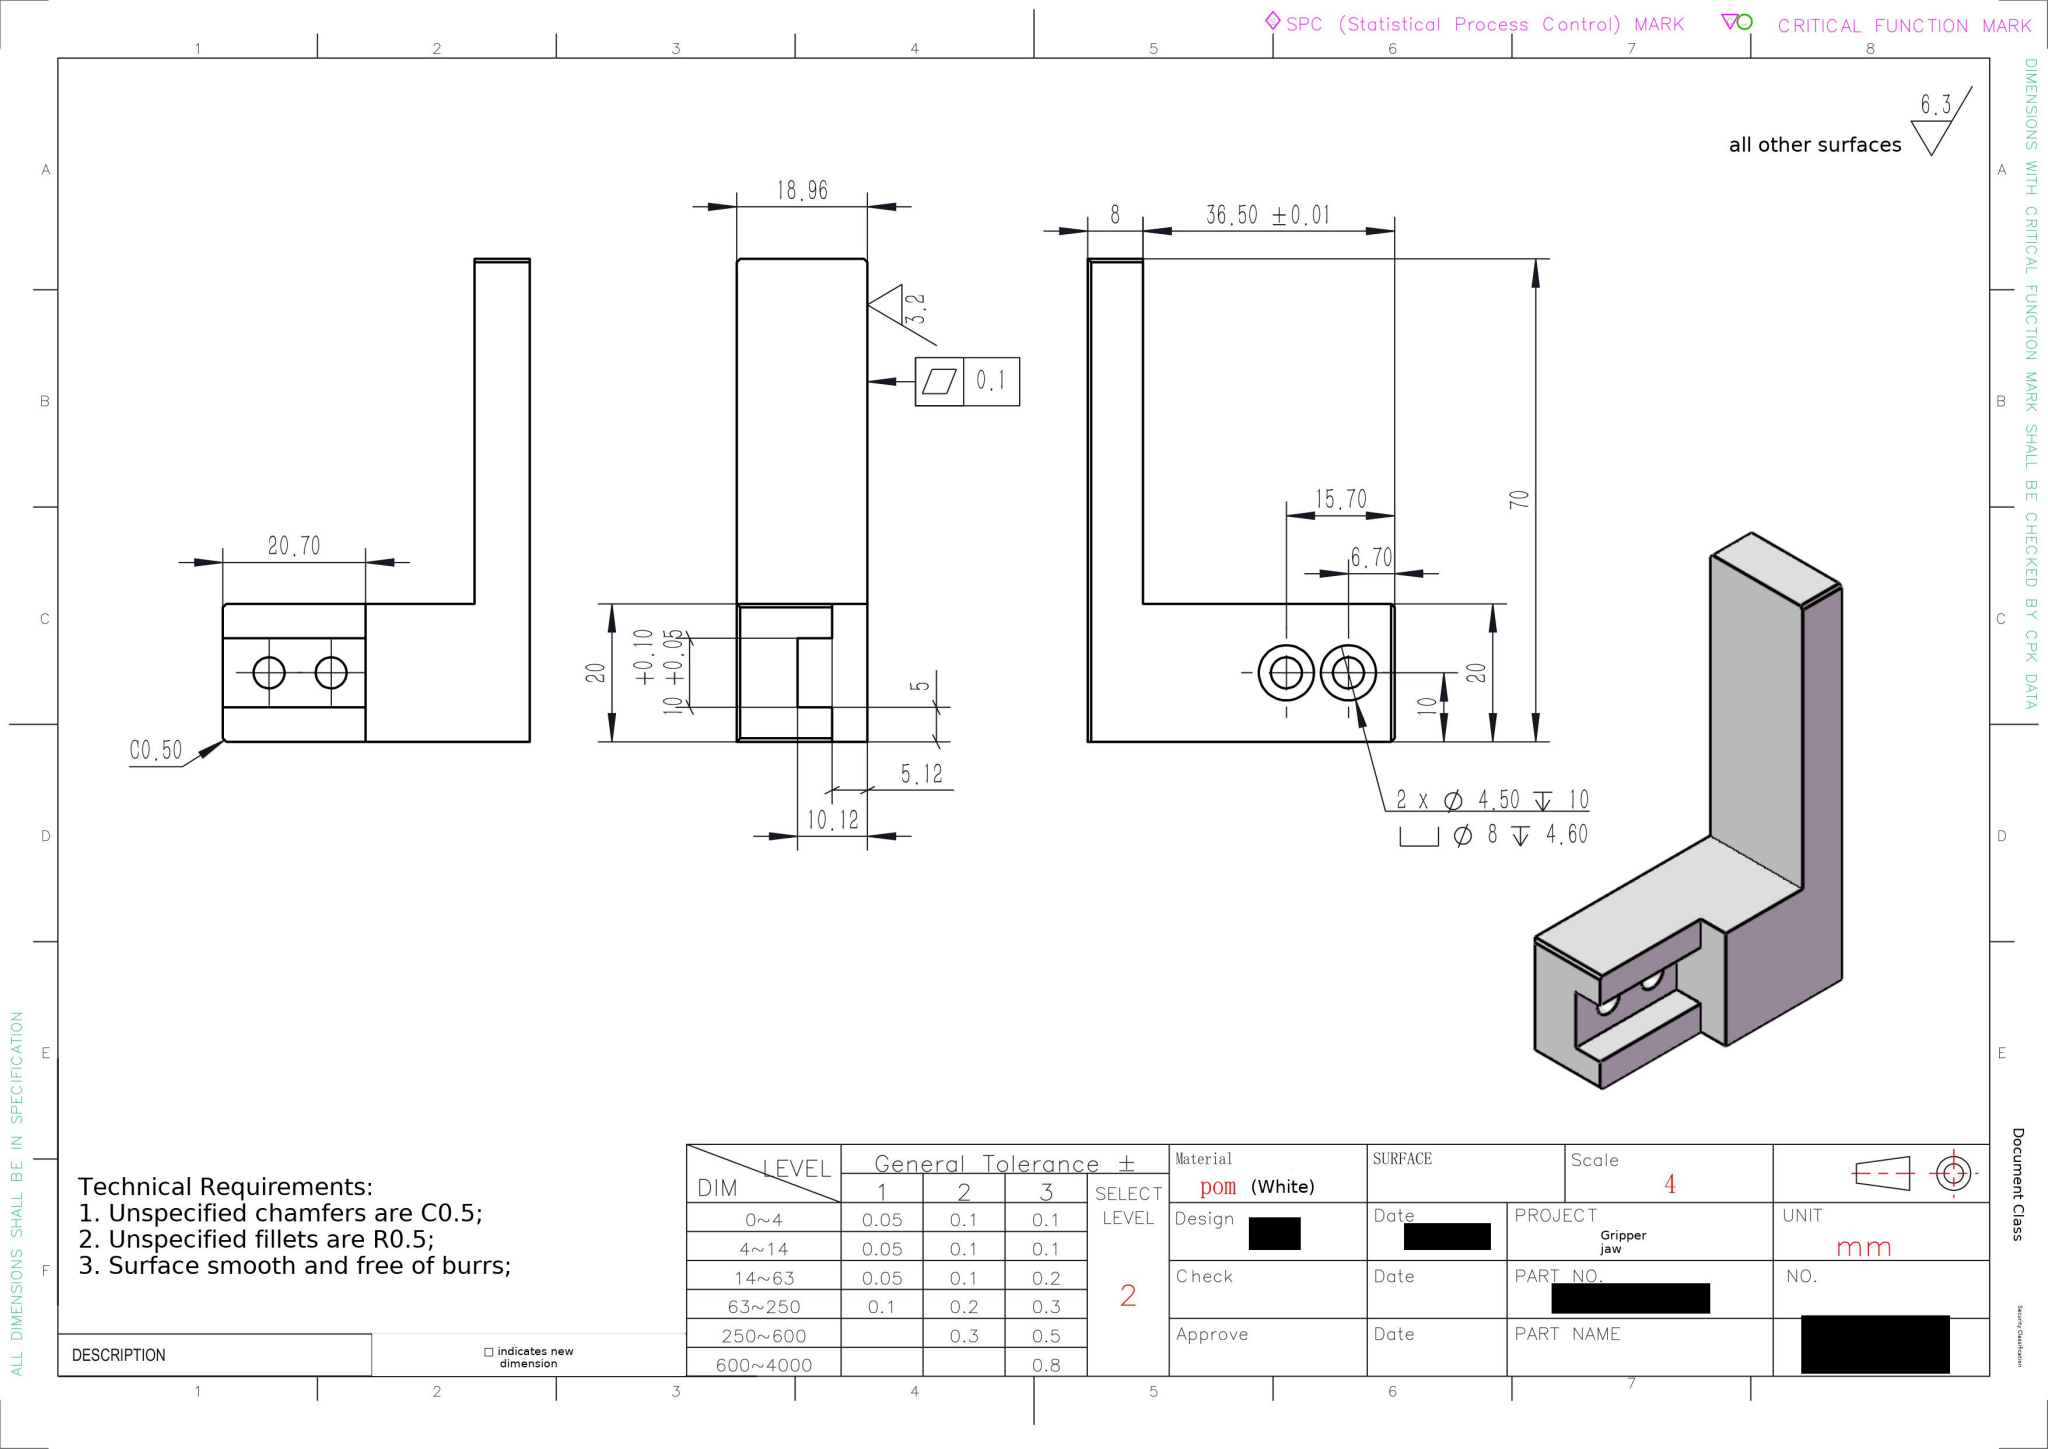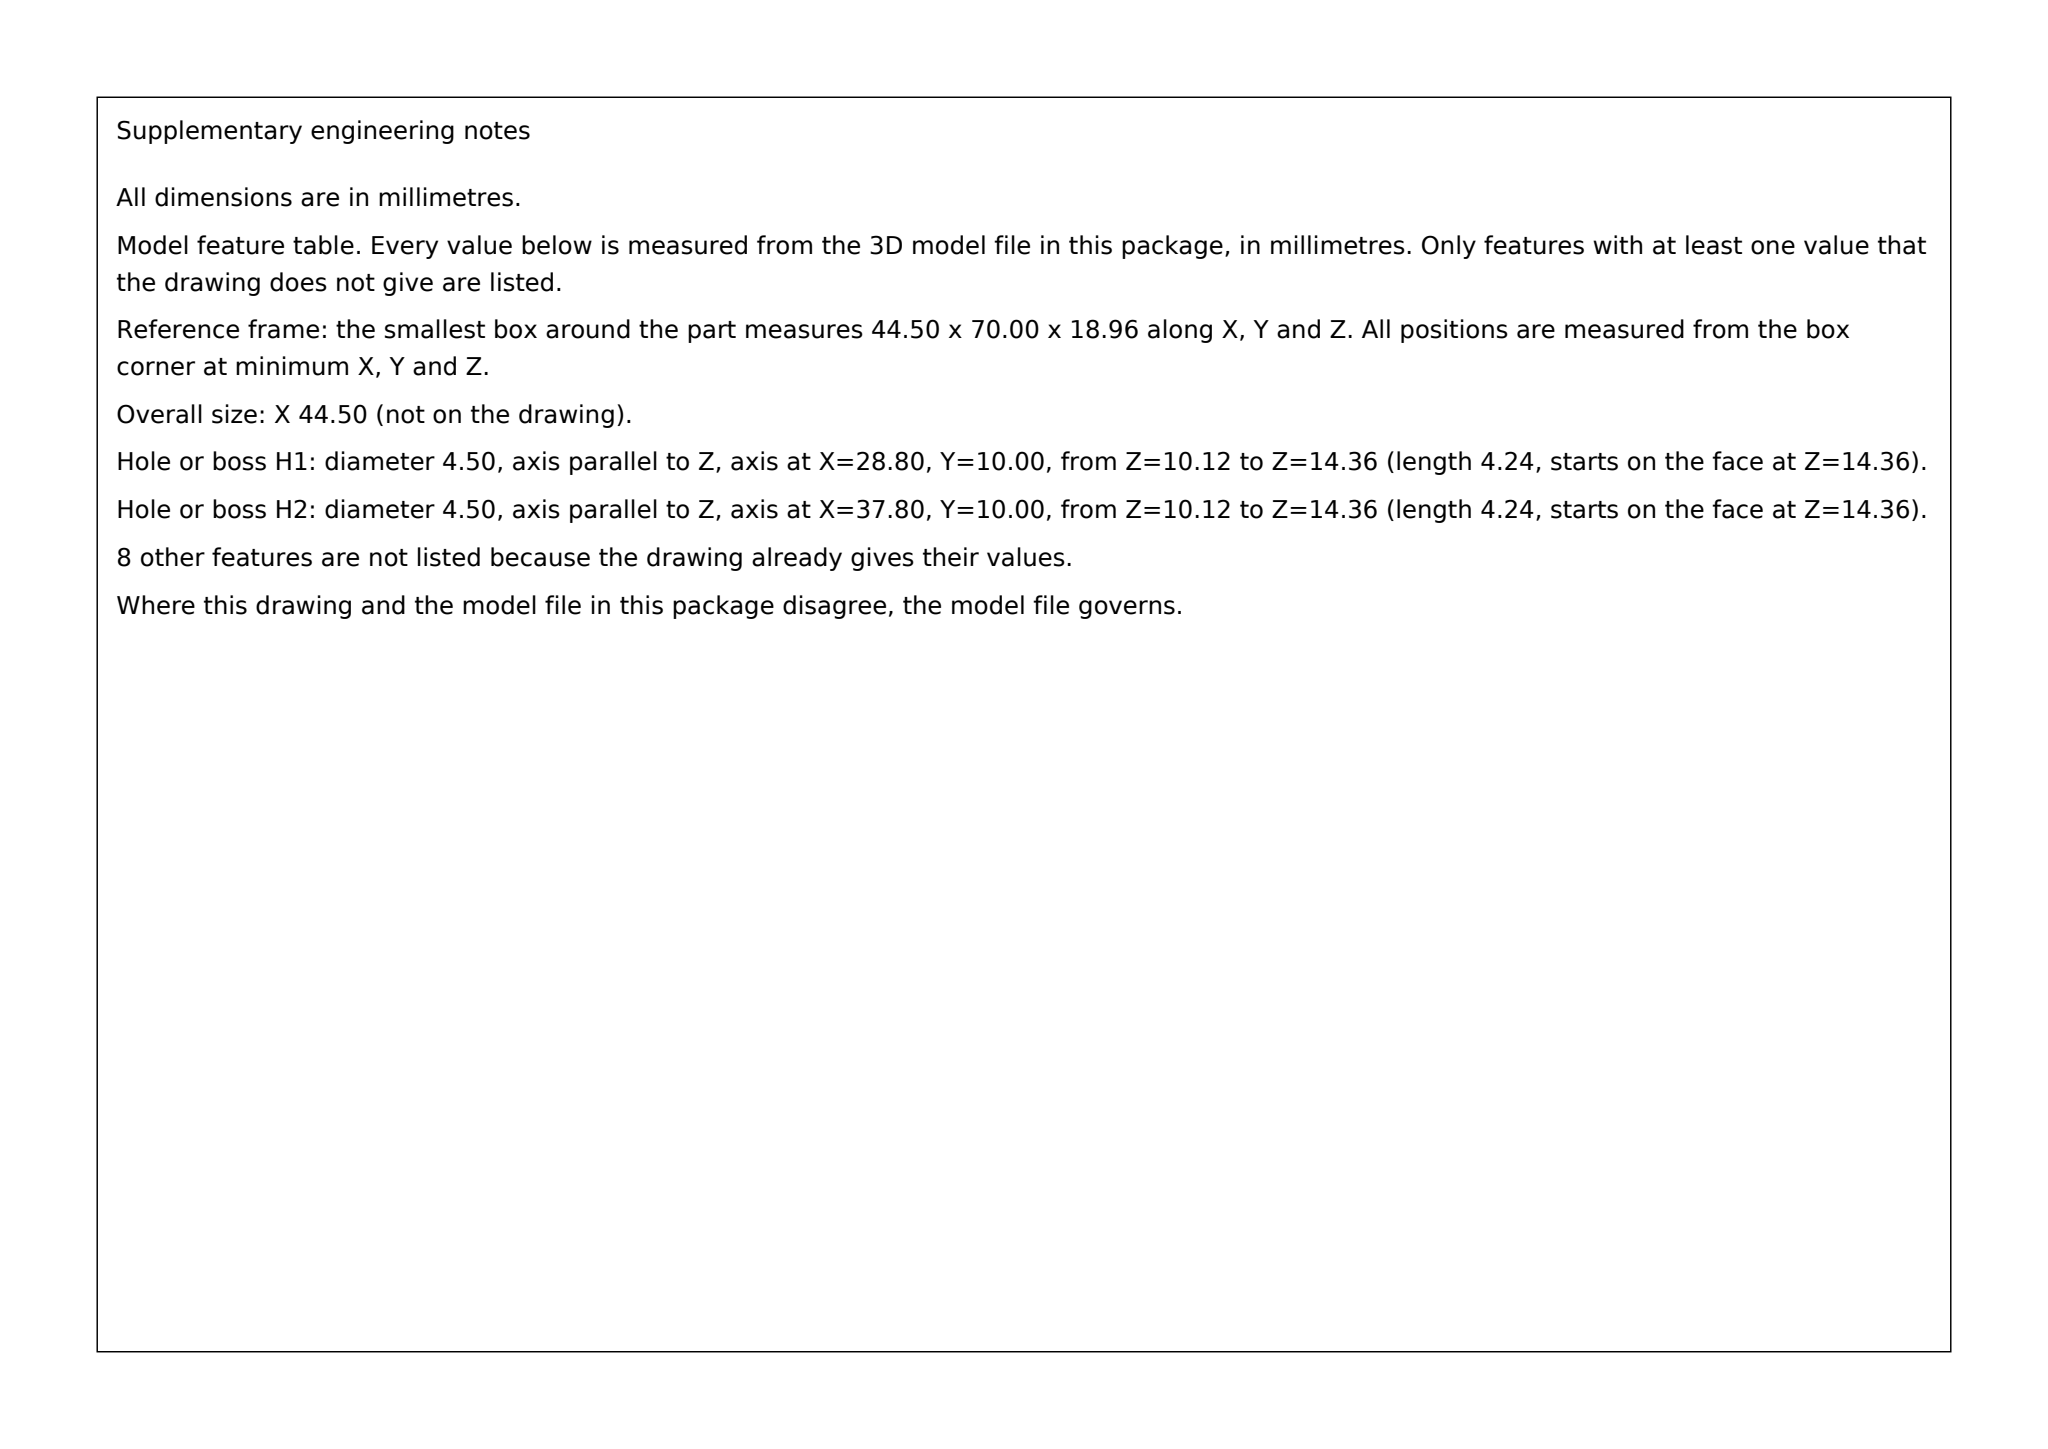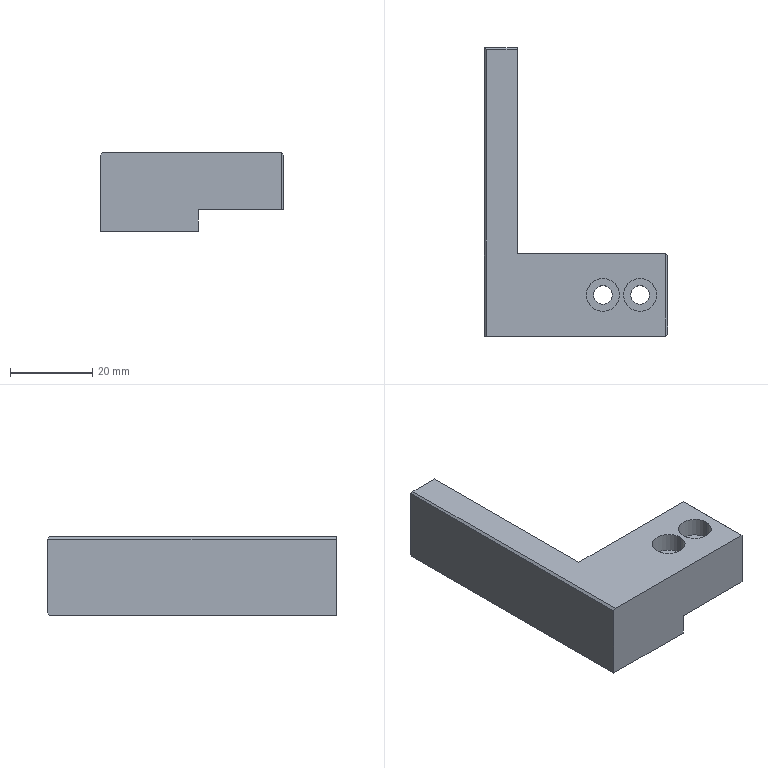Part | SolidWorks | mm | material pom (White) | 1 solid | 30 faces | box 44.5 x 70 x 18.96 mm | volume 20690 mm3 | plane 22 | cylinder 8 | commonest cylinder face diameters 8 x4 4.5 x4
build123d program:
from build123d import *

# Parameters (mm, degrees)
SKETCH1_W                                         = 50
SKETCH1_H                                         = 20
BOSS_EXTRUDE1_DEPTH                               = 44.5
SKETCH2_W                                         = 32.32
SKETCH2_H                                         = 10
CUT_EXTRUDE1_DEPTH                                = 20.7
HOLE_SIZE_ACCORDING_TO_HEXAGON_SOCKET_D           = 4.5
HOLE_SIZE_ACCORDING_TO_HEXAGON_SOCKET_DEPTH       = 10
HOLE_SIZE_ACCORDING_TO_HEXAGON_SOCKET_CBORE_D     = 8
HOLE_SIZE_ACCORDING_TO_HEXAGON_SOCKET_CBORE_DEPTH = 4.6
HOLE_SIZE_ACCORDING_TO_HEXAGON_SOCKET_TIP         = 1.352
HOLE_SIZE_ACCORDING_TO_HEXAGON_SO_2_D             = 4.5
HOLE_SIZE_ACCORDING_TO_HEXAGON_SO_2_DEPTH         = 10
HOLE_SIZE_ACCORDING_TO_HEXAGON_SO_2_CBORE_D       = 8
HOLE_SIZE_ACCORDING_TO_HEXAGON_SO_2_CBORE_DEPTH   = 4.6
HOLE_SIZE_ACCORDING_TO_HEXAGON_SO_2_TIP           = 1.352
SKETCH9_W                                         = 20.7
SKETCH9_H                                         = 22.32
CUT_EXTRUDE4_DEPTH                                = 55.82
SKETCH10_W                                        = 8
SKETCH10_H                                        = 50
BOSS_EXTRUDE2_DEPTH                               = 50
SKETCH11_W                                        = 12.08
SKETCH11_H                                        = 70
CUT_EXTRUDE5_DEPTH                                = 79.773
SKETCH13_W                                        = 44.5
SKETCH13_H                                        = 18.96
CUT_EXTRUDE7_DEPTH                                = 87.633
CHAMFER1_SIZE                                     = 0.5


with BuildPart() as part:
    # Sketch1 → Boss-Extrude1 (new body)
    with BuildSketch(Plane(origin=(0, 0, 0), x_dir=(0, 0, -1), z_dir=(1, 0, 0))):
        Rectangle(SKETCH1_W, SKETCH1_H)
    extrude(amount=BOSS_EXTRUDE1_DEPTH)

    # Sketch2 → Cut-Extrude1 (cut)
    with BuildSketch(Plane(origin=(44.5, 0, 0), x_dir=(0, 0, -1), z_dir=(1, 0, 0))):
        Rectangle(SKETCH2_W, SKETCH2_H)
    extrude(amount=-CUT_EXTRUDE1_DEPTH, mode=Mode.SUBTRACT)

    # Hole Size _ according to_ Hexagon Socket
    with Locations(Plane(origin=(0, 0, -25), x_dir=(-1, 0, 0), z_dir=(0, 0, -1))):
        with Locations((-37.8, 0), (-28.8, 0)):
            CounterBoreHole(HOLE_SIZE_ACCORDING_TO_HEXAGON_SOCKET_D / 2, HOLE_SIZE_ACCORDING_TO_HEXAGON_SOCKET_CBORE_D / 2, HOLE_SIZE_ACCORDING_TO_HEXAGON_SOCKET_CBORE_DEPTH, depth=HOLE_SIZE_ACCORDING_TO_HEXAGON_SOCKET_DEPTH)
            with Locations((0, 0, -(HOLE_SIZE_ACCORDING_TO_HEXAGON_SOCKET_DEPTH + HOLE_SIZE_ACCORDING_TO_HEXAGON_SOCKET_TIP / 2))):  # 118° drill point
                Cone(0, HOLE_SIZE_ACCORDING_TO_HEXAGON_SOCKET_D / 2, HOLE_SIZE_ACCORDING_TO_HEXAGON_SOCKET_TIP, mode=Mode.SUBTRACT)

    # Hole Size _ according to_ Hexagon So 2
    with Locations(Plane.XY.offset(25)):
        with Locations((37.8, 0), (28.8, 0)):
            CounterBoreHole(HOLE_SIZE_ACCORDING_TO_HEXAGON_SO_2_D / 2, HOLE_SIZE_ACCORDING_TO_HEXAGON_SO_2_CBORE_D / 2, HOLE_SIZE_ACCORDING_TO_HEXAGON_SO_2_CBORE_DEPTH, depth=HOLE_SIZE_ACCORDING_TO_HEXAGON_SO_2_DEPTH)
            with Locations((0, 0, -(HOLE_SIZE_ACCORDING_TO_HEXAGON_SO_2_DEPTH + HOLE_SIZE_ACCORDING_TO_HEXAGON_SO_2_TIP / 2))):  # 118° drill point
                Cone(0, HOLE_SIZE_ACCORDING_TO_HEXAGON_SO_2_D / 2, HOLE_SIZE_ACCORDING_TO_HEXAGON_SO_2_TIP, mode=Mode.SUBTRACT)

    # Sketch9 → Cut-Extrude4 (cut, through all)
    with BuildSketch(Plane(origin=(0, 10, 0), x_dir=(1, 0, 0), z_dir=(0, 1, 0))):
        with Locations((34.15, 0)):
            Rectangle(SKETCH9_W, SKETCH9_H)
    extrude(amount=-CUT_EXTRUDE4_DEPTH, mode=Mode.SUBTRACT)

    # Sketch10 → Boss-Extrude2 (add)
    with BuildSketch(Plane(origin=(0, 10, 0), x_dir=(1, 0, 0), z_dir=(0, 1, 0))):
        with Locations((4, 0)):
            Rectangle(SKETCH10_W, SKETCH10_H)
    extrude(amount=BOSS_EXTRUDE2_DEPTH)

    # Sketch11 → Cut-Extrude5 (cut, through all)
    with BuildSketch(Plane.ZY):
        with Locations((0, 25)):
            Rectangle(SKETCH11_W, SKETCH11_H)
    extrude(amount=-CUT_EXTRUDE5_DEPTH, mode=Mode.SUBTRACT)


with BuildPart() as cut_extrude5_piece_1:
    # of the separate pieces the step leaves, piece 1, a body of its own (cut_extrude5_pieces)
    add(part.part.solids().sort_by_distance((8, 10, 6.04))[0])

    # Chamfer1
    chamfer1_edges = [cut_extrude5_piece_1.edges().sort_by_distance(p)[0] for p in [
        (44.5, 0, 25),
        (4, 60, 6.04),
        (44.5, -10, 18.08),
        (0, 25, 25),
        (44.5, 10, 18.08),
        (4, 60, 25),
    ]]
    chamfer(chamfer1_edges, length=CHAMFER1_SIZE)


with BuildPart() as cut_extrude5_piece_2:
    # of the separate pieces the step leaves, piece 2, a body of its own (cut_extrude5_pieces)
    add(part.part.solids().sort_by_distance((8, 10, -25))[0])

    # Sketch13 → Cut-Extrude7 (cut, through all)
    with BuildSketch(Plane.XZ.offset(10)):
        with Locations((22.25, -15.52)):
            Rectangle(SKETCH13_W, SKETCH13_H)
    extrude(amount=-CUT_EXTRUDE7_DEPTH, mode=Mode.SUBTRACT)


solid = cut_extrude5_piece_1.part
STEP:
#1=CARTESIAN_POINT('',(33.8,-0.,20.4));
#2=VERTEX_POINT('',#1);
#3=CARTESIAN_POINT('',(41.8,-0.,20.4));
#4=VERTEX_POINT('',#3);
#5=CARTESIAN_POINT('',(37.8,-0.,20.4));
#6=DIRECTION('',(0.,0.,1.));
#7=DIRECTION('',(1.,0.,0.));
#8=AXIS2_PLACEMENT_3D('',#5,#6,#7);
#9=CIRCLE('',#8,4.);
#10=EDGE_CURVE('',#2,#4,#9,.T.);
#11=ORIENTED_EDGE('',*,*,#10,.F.);
#12=CARTESIAN_POINT('',(33.8,-0.,25.));
#13=VERTEX_POINT('',#12);
#14=CARTESIAN_POINT('',(33.8,-0.,25.));
#15=DIRECTION('',(0.,0.,1.));
#16=VECTOR('',#15,1000.);
#17=LINE('',#14,#16);
#18=EDGE_CURVE('',#2,#13,#17,.T.);
#19=ORIENTED_EDGE('',*,*,#18,.T.);
#20=CARTESIAN_POINT('',(41.8,-0.,25.));
#21=VERTEX_POINT('',#20);
#22=CARTESIAN_POINT('',(37.8,-0.,25.));
#23=DIRECTION('',(0.,0.,1.));
#24=DIRECTION('',(1.,0.,0.));
#25=AXIS2_PLACEMENT_3D('',#22,#23,#24);
#26=CIRCLE('',#25,4.);
#27=EDGE_CURVE('',#13,#21,#26,.T.);
#28=ORIENTED_EDGE('',*,*,#27,.T.);
#29=CARTESIAN_POINT('',(41.8,-0.,25.));
#30=DIRECTION('',(0.,0.,1.));
#31=VECTOR('',#30,1000.);
#32=LINE('',#29,#31);
#33=EDGE_CURVE('',#4,#21,#32,.T.);
#34=ORIENTED_EDGE('',*,*,#33,.F.);
#35=EDGE_LOOP('',(#11,#19,#28,#34));
#36=FACE_OUTER_BOUND('',#35,.T.);
#37=CARTESIAN_POINT('',(37.8,-0.,25.));
#38=DIRECTION('',(0.,0.,1.));
#39=DIRECTION('',(1.,0.,0.));
#40=AXIS2_PLACEMENT_3D('',#37,#38,#39);
#41=CYLINDRICAL_SURFACE('',#40,4.);
#42=ADVANCED_FACE('',(#36),#41,.F.);
#43=CARTESIAN_POINT('',(24.8,-0.,20.4));
#44=VERTEX_POINT('',#43);
#45=CARTESIAN_POINT('',(32.8,-0.,20.4));
#46=VERTEX_POINT('',#45);
#47=CARTESIAN_POINT('',(28.8,-0.,20.4));
#48=DIRECTION('',(0.,0.,1.));
#49=DIRECTION('',(1.,0.,0.));
#50=AXIS2_PLACEMENT_3D('',#47,#48,#49);
#51=CIRCLE('',#50,4.);
#52=EDGE_CURVE('',#44,#46,#51,.T.);
#53=ORIENTED_EDGE('',*,*,#52,.F.);
#54=CARTESIAN_POINT('',(24.8,-0.,25.));
#55=VERTEX_POINT('',#54);
#56=CARTESIAN_POINT('',(24.8,-0.,25.));
#57=DIRECTION('',(0.,0.,1.));
#58=VECTOR('',#57,1000.);
#59=LINE('',#56,#58);
#60=EDGE_CURVE('',#44,#55,#59,.T.);
#61=ORIENTED_EDGE('',*,*,#60,.T.);
#62=CARTESIAN_POINT('',(32.8,-0.,25.));
#63=VERTEX_POINT('',#62);
#64=CARTESIAN_POINT('',(28.8,-0.,25.));
#65=DIRECTION('',(0.,0.,1.));
#66=DIRECTION('',(1.,0.,0.));
#67=AXIS2_PLACEMENT_3D('',#64,#65,#66);
#68=CIRCLE('',#67,4.);
#69=EDGE_CURVE('',#55,#63,#68,.T.);
#70=ORIENTED_EDGE('',*,*,#69,.T.);
#71=CARTESIAN_POINT('',(32.8,-0.,25.));
#72=DIRECTION('',(0.,0.,1.));
#73=VECTOR('',#72,1000.);
#74=LINE('',#71,#73);
#75=EDGE_CURVE('',#46,#63,#74,.T.);
#76=ORIENTED_EDGE('',*,*,#75,.F.);
#77=EDGE_LOOP('',(#53,#61,#70,#76));
#78=FACE_OUTER_BOUND('',#77,.T.);
#79=CARTESIAN_POINT('',(28.8,-0.,25.));
#80=DIRECTION('',(0.,0.,1.));
#81=DIRECTION('',(1.,0.,0.));
#82=AXIS2_PLACEMENT_3D('',#79,#80,#81);
#83=CYLINDRICAL_SURFACE('',#82,4.);
#84=ADVANCED_FACE('',(#78),#83,.F.);
#85=CARTESIAN_POINT('',(35.55,-0.,16.16));
#86=VERTEX_POINT('',#85);
#87=CARTESIAN_POINT('',(40.05,-0.,16.16));
#88=VERTEX_POINT('',#87);
#89=CARTESIAN_POINT('',(37.8,-0.,16.16));
#90=DIRECTION('',(0.,0.,1.));
#91=DIRECTION('',(1.,0.,0.));
#92=AXIS2_PLACEMENT_3D('',#89,#90,#91);
#93=CIRCLE('',#92,2.25);
#94=EDGE_CURVE('',#86,#88,#93,.T.);
#95=ORIENTED_EDGE('',*,*,#94,.F.);
#96=CARTESIAN_POINT('',(35.55,-0.,20.4));
#97=VERTEX_POINT('',#96);
#98=CARTESIAN_POINT('',(35.55,-0.,25.));
#99=DIRECTION('',(0.,0.,1.));
#100=VECTOR('',#99,1000.);
#101=LINE('',#98,#100);
#102=EDGE_CURVE('',#86,#97,#101,.T.);
#103=ORIENTED_EDGE('',*,*,#102,.T.);
#104=CARTESIAN_POINT('',(40.05,-0.,20.4));
#105=VERTEX_POINT('',#104);
#106=CARTESIAN_POINT('',(37.8,-0.,20.4));
#107=DIRECTION('',(0.,0.,1.));
#108=DIRECTION('',(1.,0.,0.));
#109=AXIS2_PLACEMENT_3D('',#106,#107,#108);
#110=CIRCLE('',#109,2.25);
#111=EDGE_CURVE('',#97,#105,#110,.T.);
#112=ORIENTED_EDGE('',*,*,#111,.T.);
#113=CARTESIAN_POINT('',(40.05,-0.,25.));
#114=DIRECTION('',(0.,0.,1.));
#115=VECTOR('',#114,1000.);
#116=LINE('',#113,#115);
#117=EDGE_CURVE('',#88,#105,#116,.T.);
#118=ORIENTED_EDGE('',*,*,#117,.F.);
#119=EDGE_LOOP('',(#95,#103,#112,#118));
#120=FACE_OUTER_BOUND('',#119,.T.);
#121=CARTESIAN_POINT('',(37.8,-0.,25.));
#122=DIRECTION('',(0.,0.,1.));
#123=DIRECTION('',(1.,0.,0.));
#124=AXIS2_PLACEMENT_3D('',#121,#122,#123);
#125=CYLINDRICAL_SURFACE('',#124,2.25);
#126=ADVANCED_FACE('',(#120),#125,.F.);
#127=CARTESIAN_POINT('',(26.55,-0.,16.16));
#128=VERTEX_POINT('',#127);
#129=CARTESIAN_POINT('',(31.05,-0.,16.16));
#130=VERTEX_POINT('',#129);
#131=CARTESIAN_POINT('',(28.8,-0.,16.16));
#132=DIRECTION('',(0.,0.,1.));
#133=DIRECTION('',(1.,0.,0.));
#134=AXIS2_PLACEMENT_3D('',#131,#132,#133);
#135=CIRCLE('',#134,2.25);
#136=EDGE_CURVE('',#128,#130,#135,.T.);
#137=ORIENTED_EDGE('',*,*,#136,.F.);
#138=CARTESIAN_POINT('',(26.55,-0.,20.4));
#139=VERTEX_POINT('',#138);
#140=CARTESIAN_POINT('',(26.55,-0.,25.));
#141=DIRECTION('',(0.,0.,1.));
#142=VECTOR('',#141,1000.);
#143=LINE('',#140,#142);
#144=EDGE_CURVE('',#128,#139,#143,.T.);
#145=ORIENTED_EDGE('',*,*,#144,.T.);
#146=CARTESIAN_POINT('',(31.05,-0.,20.4));
#147=VERTEX_POINT('',#146);
#148=CARTESIAN_POINT('',(28.8,-0.,20.4));
#149=DIRECTION('',(0.,0.,1.));
#150=DIRECTION('',(1.,0.,0.));
#151=AXIS2_PLACEMENT_3D('',#148,#149,#150);
#152=CIRCLE('',#151,2.25);
#153=EDGE_CURVE('',#139,#147,#152,.T.);
#154=ORIENTED_EDGE('',*,*,#153,.T.);
#155=CARTESIAN_POINT('',(31.05,-0.,25.));
#156=DIRECTION('',(0.,0.,1.));
#157=VECTOR('',#156,1000.);
#158=LINE('',#155,#157);
#159=EDGE_CURVE('',#130,#147,#158,.T.);
#160=ORIENTED_EDGE('',*,*,#159,.F.);
#161=EDGE_LOOP('',(#137,#145,#154,#160));
#162=FACE_OUTER_BOUND('',#161,.T.);
#163=CARTESIAN_POINT('',(28.8,-0.,25.));
#164=DIRECTION('',(0.,0.,1.));
#165=DIRECTION('',(1.,0.,0.));
#166=AXIS2_PLACEMENT_3D('',#163,#164,#165);
#167=CYLINDRICAL_SURFACE('',#166,2.25);
#168=ADVANCED_FACE('',(#162),#167,.F.);
#169=CARTESIAN_POINT('',(28.8,-0.,20.4));
#170=DIRECTION('',(0.,0.,1.));
#171=DIRECTION('',(1.,0.,0.));
#172=AXIS2_PLACEMENT_3D('',#169,#170,#171);
#173=CIRCLE('',#172,2.25);
#174=EDGE_CURVE('',#147,#139,#173,.T.);
#175=ORIENTED_EDGE('',*,*,#174,.F.);
#176=ORIENTED_EDGE('',*,*,#153,.F.);
#177=EDGE_LOOP('',(#175,#176));
#178=FACE_BOUND('',#177,.T.);
#179=CARTESIAN_POINT('',(28.8,-0.,20.4));
#180=DIRECTION('',(0.,0.,1.));
#181=DIRECTION('',(1.,0.,0.));
#182=AXIS2_PLACEMENT_3D('',#179,#180,#181);
#183=CIRCLE('',#182,4.);
#184=EDGE_CURVE('',#46,#44,#183,.T.);
#185=ORIENTED_EDGE('',*,*,#184,.T.);
#186=ORIENTED_EDGE('',*,*,#52,.T.);
#187=EDGE_LOOP('',(#185,#186));
#188=FACE_OUTER_BOUND('',#187,.T.);
#189=CARTESIAN_POINT('',(31.05,-0.,20.4));
#190=DIRECTION('',(0.,0.,-1.));
#191=DIRECTION('',(-1.,0.,0.));
#192=AXIS2_PLACEMENT_3D('',#189,#190,#191);
#193=PLANE('',#192);
#194=ADVANCED_FACE('',(#178,#188),#193,.F.);
#195=CARTESIAN_POINT('',(37.8,-0.,20.4));
#196=DIRECTION('',(0.,0.,1.));
#197=DIRECTION('',(1.,0.,0.));
#198=AXIS2_PLACEMENT_3D('',#195,#196,#197);
#199=CIRCLE('',#198,2.25);
#200=EDGE_CURVE('',#105,#97,#199,.T.);
#201=ORIENTED_EDGE('',*,*,#200,.F.);
#202=ORIENTED_EDGE('',*,*,#111,.F.);
#203=EDGE_LOOP('',(#201,#202));
#204=FACE_BOUND('',#203,.T.);
#205=CARTESIAN_POINT('',(37.8,-0.,20.4));
#206=DIRECTION('',(0.,0.,1.));
#207=DIRECTION('',(1.,0.,0.));
#208=AXIS2_PLACEMENT_3D('',#205,#206,#207);
#209=CIRCLE('',#208,4.);
#210=EDGE_CURVE('',#4,#2,#209,.T.);
#211=ORIENTED_EDGE('',*,*,#210,.T.);
#212=ORIENTED_EDGE('',*,*,#10,.T.);
#213=EDGE_LOOP('',(#211,#212));
#214=FACE_OUTER_BOUND('',#213,.T.);
#215=CARTESIAN_POINT('',(40.05,-0.,20.4));
#216=DIRECTION('',(0.,0.,-1.));
#217=DIRECTION('',(-1.,0.,0.));
#218=AXIS2_PLACEMENT_3D('',#215,#216,#217);
#219=PLANE('',#218);
#220=ADVANCED_FACE('',(#204,#214),#219,.F.);
#221=ORIENTED_EDGE('',*,*,#144,.F.);
#222=CARTESIAN_POINT('',(28.8,-0.,16.16));
#223=DIRECTION('',(0.,0.,1.));
#224=DIRECTION('',(1.,0.,0.));
#225=AXIS2_PLACEMENT_3D('',#222,#223,#224);
#226=CIRCLE('',#225,2.25);
#227=EDGE_CURVE('',#130,#128,#226,.T.);
#228=ORIENTED_EDGE('',*,*,#227,.F.);
#229=ORIENTED_EDGE('',*,*,#159,.T.);
#230=ORIENTED_EDGE('',*,*,#174,.T.);
#231=EDGE_LOOP('',(#221,#228,#229,#230));
#232=FACE_OUTER_BOUND('',#231,.T.);
#233=CARTESIAN_POINT('',(28.8,-0.,25.));
#234=DIRECTION('',(0.,0.,1.));
#235=DIRECTION('',(1.,0.,0.));
#236=AXIS2_PLACEMENT_3D('',#233,#234,#235);
#237=CYLINDRICAL_SURFACE('',#236,2.25);
#238=ADVANCED_FACE('',(#232),#237,.F.);
#239=ORIENTED_EDGE('',*,*,#102,.F.);
#240=CARTESIAN_POINT('',(37.8,-0.,16.16));
#241=DIRECTION('',(0.,0.,1.));
#242=DIRECTION('',(1.,0.,0.));
#243=AXIS2_PLACEMENT_3D('',#240,#241,#242);
#244=CIRCLE('',#243,2.25);
#245=EDGE_CURVE('',#88,#86,#244,.T.);
#246=ORIENTED_EDGE('',*,*,#245,.F.);
#247=ORIENTED_EDGE('',*,*,#117,.T.);
#248=ORIENTED_EDGE('',*,*,#200,.T.);
#249=EDGE_LOOP('',(#239,#246,#247,#248));
#250=FACE_OUTER_BOUND('',#249,.T.);
#251=CARTESIAN_POINT('',(37.8,-0.,25.));
#252=DIRECTION('',(0.,0.,1.));
#253=DIRECTION('',(1.,0.,0.));
#254=AXIS2_PLACEMENT_3D('',#251,#252,#253);
#255=CYLINDRICAL_SURFACE('',#254,2.25);
#256=ADVANCED_FACE('',(#250),#255,.F.);
#257=ORIENTED_EDGE('',*,*,#60,.F.);
#258=ORIENTED_EDGE('',*,*,#184,.F.);
#259=ORIENTED_EDGE('',*,*,#75,.T.);
#260=CARTESIAN_POINT('',(28.8,-0.,25.));
#261=DIRECTION('',(0.,0.,1.));
#262=DIRECTION('',(1.,0.,0.));
#263=AXIS2_PLACEMENT_3D('',#260,#261,#262);
#264=CIRCLE('',#263,4.);
#265=EDGE_CURVE('',#63,#55,#264,.T.);
#266=ORIENTED_EDGE('',*,*,#265,.T.);
#267=EDGE_LOOP('',(#257,#258,#259,#266));
#268=FACE_OUTER_BOUND('',#267,.T.);
#269=CARTESIAN_POINT('',(28.8,-0.,25.));
#270=DIRECTION('',(0.,0.,1.));
#271=DIRECTION('',(1.,0.,0.));
#272=AXIS2_PLACEMENT_3D('',#269,#270,#271);
#273=CYLINDRICAL_SURFACE('',#272,4.);
#274=ADVANCED_FACE('',(#268),#273,.F.);
#275=ORIENTED_EDGE('',*,*,#18,.F.);
#276=ORIENTED_EDGE('',*,*,#210,.F.);
#277=ORIENTED_EDGE('',*,*,#33,.T.);
#278=CARTESIAN_POINT('',(37.8,-0.,25.));
#279=DIRECTION('',(0.,0.,1.));
#280=DIRECTION('',(1.,0.,0.));
#281=AXIS2_PLACEMENT_3D('',#278,#279,#280);
#282=CIRCLE('',#281,4.);
#283=EDGE_CURVE('',#21,#13,#282,.T.);
#284=ORIENTED_EDGE('',*,*,#283,.T.);
#285=EDGE_LOOP('',(#275,#276,#277,#284));
#286=FACE_OUTER_BOUND('',#285,.T.);
#287=CARTESIAN_POINT('',(37.8,-0.,25.));
#288=DIRECTION('',(0.,0.,1.));
#289=DIRECTION('',(1.,0.,0.));
#290=AXIS2_PLACEMENT_3D('',#287,#288,#289);
#291=CYLINDRICAL_SURFACE('',#290,4.);
#292=ADVANCED_FACE('',(#286),#291,.F.);
#293=CARTESIAN_POINT('',(44.5,9.5,24.5));
#294=VERTEX_POINT('',#293);
#295=CARTESIAN_POINT('',(44.5,-9.5,24.5));
#296=VERTEX_POINT('',#295);
#297=CARTESIAN_POINT('',(44.5,-10.,24.5));
#298=DIRECTION('',(0.,-1.,-0.));
#299=VECTOR('',#298,1000.);
#300=LINE('',#297,#299);
#301=EDGE_CURVE('',#294,#296,#300,.T.);
#302=ORIENTED_EDGE('',*,*,#301,.T.);
#303=CARTESIAN_POINT('',(44.5,-9.5,11.16));
#304=VERTEX_POINT('',#303);
#305=CARTESIAN_POINT('',(44.5,-9.5,11.16));
#306=DIRECTION('',(0.,0.,-1.));
#307=VECTOR('',#306,1000.);
#308=LINE('',#305,#307);
#309=EDGE_CURVE('',#296,#304,#308,.T.);
#310=ORIENTED_EDGE('',*,*,#309,.T.);
#311=CARTESIAN_POINT('',(44.5,-5.,11.16));
#312=VERTEX_POINT('',#311);
#313=CARTESIAN_POINT('',(44.5,-10.,11.16));
#314=DIRECTION('',(0.,1.,0.));
#315=VECTOR('',#314,1000.);
#316=LINE('',#313,#315);
#317=EDGE_CURVE('',#304,#312,#316,.T.);
#318=ORIENTED_EDGE('',*,*,#317,.T.);
#319=CARTESIAN_POINT('',(44.5,-5.,16.16));
#320=VERTEX_POINT('',#319);
#321=CARTESIAN_POINT('',(44.5,-5.,16.16));
#322=DIRECTION('',(0.,0.,-1.));
#323=VECTOR('',#322,1000.);
#324=LINE('',#321,#323);
#325=EDGE_CURVE('',#320,#312,#324,.T.);
#326=ORIENTED_EDGE('',*,*,#325,.F.);
#327=CARTESIAN_POINT('',(44.5,5.,16.16));
#328=VERTEX_POINT('',#327);
#329=CARTESIAN_POINT('',(44.5,5.,16.16));
#330=DIRECTION('',(0.,-1.,0.));
#331=VECTOR('',#330,1000.);
#332=LINE('',#329,#331);
#333=EDGE_CURVE('',#328,#320,#332,.T.);
#334=ORIENTED_EDGE('',*,*,#333,.F.);
#335=CARTESIAN_POINT('',(44.5,5.,11.16));
#336=VERTEX_POINT('',#335);
#337=CARTESIAN_POINT('',(44.5,5.,16.16));
#338=DIRECTION('',(0.,0.,1.));
#339=VECTOR('',#338,1000.);
#340=LINE('',#337,#339);
#341=EDGE_CURVE('',#336,#328,#340,.T.);
#342=ORIENTED_EDGE('',*,*,#341,.F.);
#343=CARTESIAN_POINT('',(44.5,9.5,11.16));
#344=VERTEX_POINT('',#343);
#345=CARTESIAN_POINT('',(44.5,-10.,11.16));
#346=DIRECTION('',(0.,1.,0.));
#347=VECTOR('',#346,1000.);
#348=LINE('',#345,#347);
#349=EDGE_CURVE('',#336,#344,#348,.T.);
#350=ORIENTED_EDGE('',*,*,#349,.T.);
#351=CARTESIAN_POINT('',(44.5,9.5,25.));
#352=DIRECTION('',(0.,0.,1.));
#353=VECTOR('',#352,1000.);
#354=LINE('',#351,#353);
#355=EDGE_CURVE('',#344,#294,#354,.T.);
#356=ORIENTED_EDGE('',*,*,#355,.T.);
#357=EDGE_LOOP('',(#302,#310,#318,#326,#334,#342,#350,#356));
#358=FACE_OUTER_BOUND('',#357,.T.);
#359=CARTESIAN_POINT('',(44.5,0.,0.));
#360=DIRECTION('',(1.,0.,0.));
#361=DIRECTION('',(0.,0.,-1.));
#362=AXIS2_PLACEMENT_3D('',#359,#360,#361);
#363=PLANE('',#362);
#364=ADVANCED_FACE('',(#358),#363,.T.);
#365=ORIENTED_EDGE('',*,*,#317,.F.);
#366=CARTESIAN_POINT('',(44.,-10.,11.16));
#367=VERTEX_POINT('',#366);
#368=CARTESIAN_POINT('',(44.5,-9.5,11.16));
#369=DIRECTION('',(-0.7071,-0.7071,-0.));
#370=VECTOR('',#369,1000.);
#371=LINE('',#368,#370);
#372=EDGE_CURVE('',#304,#367,#371,.T.);
#373=ORIENTED_EDGE('',*,*,#372,.T.);
#374=CARTESIAN_POINT('',(23.8,-10.,11.16));
#375=VERTEX_POINT('',#374);
#376=CARTESIAN_POINT('',(44.5,-10.,11.16));
#377=DIRECTION('',(1.,0.,0.));
#378=VECTOR('',#377,1000.);
#379=LINE('',#376,#378);
#380=EDGE_CURVE('',#375,#367,#379,.T.);
#381=ORIENTED_EDGE('',*,*,#380,.F.);
#382=CARTESIAN_POINT('',(23.8,-5.,11.16));
#383=VERTEX_POINT('',#382);
#384=CARTESIAN_POINT('',(23.8,-10.,11.16));
#385=DIRECTION('',(0.,1.,0.));
#386=VECTOR('',#385,1000.);
#387=LINE('',#384,#386);
#388=EDGE_CURVE('',#375,#383,#387,.T.);
#389=ORIENTED_EDGE('',*,*,#388,.T.);
#390=CARTESIAN_POINT('',(23.8,-5.,11.16));
#391=DIRECTION('',(-1.,0.,-0.));
#392=VECTOR('',#391,1000.);
#393=LINE('',#390,#392);
#394=EDGE_CURVE('',#312,#383,#393,.T.);
#395=ORIENTED_EDGE('',*,*,#394,.F.);
#396=EDGE_LOOP('',(#365,#373,#381,#389,#395));
#397=FACE_OUTER_BOUND('',#396,.T.);
#398=CARTESIAN_POINT('',(44.5,-10.,11.16));
#399=DIRECTION('',(-0.,0.,1.));
#400=DIRECTION('',(1.,0.,0.));
#401=AXIS2_PLACEMENT_3D('',#398,#399,#400);
#402=PLANE('',#401);
#403=ADVANCED_FACE('',(#397),#402,.F.);
#404=ORIENTED_EDGE('',*,*,#325,.T.);
#405=ORIENTED_EDGE('',*,*,#394,.T.);
#406=CARTESIAN_POINT('',(23.8,-5.,16.16));
#407=VERTEX_POINT('',#406);
#408=CARTESIAN_POINT('',(23.8,-5.,16.16));
#409=DIRECTION('',(0.,0.,-1.));
#410=VECTOR('',#409,1000.);
#411=LINE('',#408,#410);
#412=EDGE_CURVE('',#407,#383,#411,.T.);
#413=ORIENTED_EDGE('',*,*,#412,.F.);
#414=CARTESIAN_POINT('',(23.8,-5.,16.16));
#415=DIRECTION('',(1.,0.,0.));
#416=VECTOR('',#415,1000.);
#417=LINE('',#414,#416);
#418=EDGE_CURVE('',#407,#320,#417,.T.);
#419=ORIENTED_EDGE('',*,*,#418,.T.);
#420=EDGE_LOOP('',(#404,#405,#413,#419));
#421=FACE_OUTER_BOUND('',#420,.T.);
#422=CARTESIAN_POINT('',(23.8,-5.,16.16));
#423=DIRECTION('',(0.,-1.,0.));
#424=DIRECTION('',(0.,0.,-1.));
#425=AXIS2_PLACEMENT_3D('',#422,#423,#424);
#426=PLANE('',#425);
#427=ADVANCED_FACE('',(#421),#426,.F.);
#428=ORIENTED_EDGE('',*,*,#245,.T.);
#429=ORIENTED_EDGE('',*,*,#94,.T.);
#430=EDGE_LOOP('',(#428,#429));
#431=FACE_BOUND('',#430,.T.);
#432=ORIENTED_EDGE('',*,*,#227,.T.);
#433=ORIENTED_EDGE('',*,*,#136,.T.);
#434=EDGE_LOOP('',(#432,#433));
#435=FACE_BOUND('',#434,.T.);
#436=ORIENTED_EDGE('',*,*,#333,.T.);
#437=ORIENTED_EDGE('',*,*,#418,.F.);
#438=CARTESIAN_POINT('',(23.8,5.,16.16));
#439=VERTEX_POINT('',#438);
#440=CARTESIAN_POINT('',(23.8,5.,16.16));
#441=DIRECTION('',(0.,-1.,0.));
#442=VECTOR('',#441,1000.);
#443=LINE('',#440,#442);
#444=EDGE_CURVE('',#439,#407,#443,.T.);
#445=ORIENTED_EDGE('',*,*,#444,.F.);
#446=CARTESIAN_POINT('',(23.8,5.,16.16));
#447=DIRECTION('',(1.,0.,0.));
#448=VECTOR('',#447,1000.);
#449=LINE('',#446,#448);
#450=EDGE_CURVE('',#439,#328,#449,.T.);
#451=ORIENTED_EDGE('',*,*,#450,.T.);
#452=EDGE_LOOP('',(#436,#437,#445,#451));
#453=FACE_OUTER_BOUND('',#452,.T.);
#454=CARTESIAN_POINT('',(23.8,5.,16.16));
#455=DIRECTION('',(0.,0.,1.));
#456=DIRECTION('',(1.,0.,0.));
#457=AXIS2_PLACEMENT_3D('',#454,#455,#456);
#458=PLANE('',#457);
#459=ADVANCED_FACE('',(#431,#435,#453),#458,.F.);
#460=CARTESIAN_POINT('',(23.8,5.,11.16));
#461=VERTEX_POINT('',#460);
#462=CARTESIAN_POINT('',(23.8,5.,16.16));
#463=DIRECTION('',(0.,0.,1.));
#464=VECTOR('',#463,1000.);
#465=LINE('',#462,#464);
#466=EDGE_CURVE('',#461,#439,#465,.T.);
#467=ORIENTED_EDGE('',*,*,#466,.F.);
#468=CARTESIAN_POINT('',(23.8,5.,11.16));
#469=DIRECTION('',(1.,0.,0.));
#470=VECTOR('',#469,1000.);
#471=LINE('',#468,#470);
#472=EDGE_CURVE('',#461,#336,#471,.T.);
#473=ORIENTED_EDGE('',*,*,#472,.T.);
#474=ORIENTED_EDGE('',*,*,#341,.T.);
#475=ORIENTED_EDGE('',*,*,#450,.F.);
#476=EDGE_LOOP('',(#467,#473,#474,#475));
#477=FACE_OUTER_BOUND('',#476,.T.);
#478=CARTESIAN_POINT('',(23.8,5.,16.16));
#479=DIRECTION('',(0.,1.,0.));
#480=DIRECTION('',(0.,0.,1.));
#481=AXIS2_PLACEMENT_3D('',#478,#479,#480);
#482=PLANE('',#481);
#483=ADVANCED_FACE('',(#477),#482,.F.);
#484=CARTESIAN_POINT('',(23.8,10.,11.16));
#485=VERTEX_POINT('',#484);
#486=CARTESIAN_POINT('',(44.,10.,11.16));
#487=VERTEX_POINT('',#486);
#488=CARTESIAN_POINT('',(44.5,10.,11.16));
#489=DIRECTION('',(1.,0.,0.));
#490=VECTOR('',#489,1000.);
#491=LINE('',#488,#490);
#492=EDGE_CURVE('',#485,#487,#491,.T.);
#493=ORIENTED_EDGE('',*,*,#492,.T.);
#494=CARTESIAN_POINT('',(44.5,9.5,11.16));
#495=DIRECTION('',(0.7071,-0.7071,0.));
#496=VECTOR('',#495,1000.);
#497=LINE('',#494,#496);
#498=EDGE_CURVE('',#487,#344,#497,.T.);
#499=ORIENTED_EDGE('',*,*,#498,.T.);
#500=ORIENTED_EDGE('',*,*,#349,.F.);
#501=ORIENTED_EDGE('',*,*,#472,.F.);
#502=CARTESIAN_POINT('',(23.8,-10.,11.16));
#503=DIRECTION('',(0.,1.,0.));
#504=VECTOR('',#503,1000.);
#505=LINE('',#502,#504);
#506=EDGE_CURVE('',#461,#485,#505,.T.);
#507=ORIENTED_EDGE('',*,*,#506,.T.);
#508=EDGE_LOOP('',(#493,#499,#500,#501,#507));
#509=FACE_OUTER_BOUND('',#508,.T.);
#510=CARTESIAN_POINT('',(44.5,-10.,11.16));
#511=DIRECTION('',(-0.,0.,1.));
#512=DIRECTION('',(1.,0.,0.));
#513=AXIS2_PLACEMENT_3D('',#510,#511,#512);
#514=PLANE('',#513);
#515=ADVANCED_FACE('',(#509),#514,.F.);
#516=ORIENTED_EDGE('',*,*,#283,.F.);
#517=ORIENTED_EDGE('',*,*,#27,.F.);
#518=EDGE_LOOP('',(#516,#517));
#519=FACE_BOUND('',#518,.T.);
#520=ORIENTED_EDGE('',*,*,#265,.F.);
#521=ORIENTED_EDGE('',*,*,#69,.F.);
#522=EDGE_LOOP('',(#520,#521));
#523=FACE_BOUND('',#522,.T.);
#524=CARTESIAN_POINT('',(44.,-10.,25.));
#525=VERTEX_POINT('',#524);
#526=CARTESIAN_POINT('',(0.5,-10.,25.));
#527=VERTEX_POINT('',#526);
#528=CARTESIAN_POINT('',(44.5,-10.,25.));
#529=DIRECTION('',(-1.,0.,0.));
#530=VECTOR('',#529,1000.);
#531=LINE('',#528,#530);
#532=EDGE_CURVE('',#525,#527,#531,.T.);
#533=ORIENTED_EDGE('',*,*,#532,.F.);
#534=CARTESIAN_POINT('',(44.,10.,25.));
#535=VERTEX_POINT('',#534);
#536=CARTESIAN_POINT('',(44.,10.,25.));
#537=DIRECTION('',(0.,1.,0.));
#538=VECTOR('',#537,1000.);
#539=LINE('',#536,#538);
#540=EDGE_CURVE('',#525,#535,#539,.T.);
#541=ORIENTED_EDGE('',*,*,#540,.T.);
#542=CARTESIAN_POINT('',(8.,10.,25.));
#543=VERTEX_POINT('',#542);
#544=CARTESIAN_POINT('',(44.5,10.,25.));
#545=DIRECTION('',(-1.,0.,0.));
#546=VECTOR('',#545,1000.);
#547=LINE('',#544,#546);
#548=EDGE_CURVE('',#535,#543,#547,.T.);
#549=ORIENTED_EDGE('',*,*,#548,.T.);
#550=CARTESIAN_POINT('',(8.,59.5,25.));
#551=VERTEX_POINT('',#550);
#552=CARTESIAN_POINT('',(8.,60.,25.));
#553=DIRECTION('',(0.,-1.,0.));
#554=VECTOR('',#553,1000.);
#555=LINE('',#552,#554);
#556=EDGE_CURVE('',#551,#543,#555,.T.);
#557=ORIENTED_EDGE('',*,*,#556,.F.);
#558=CARTESIAN_POINT('',(0.5,59.5,25.));
#559=VERTEX_POINT('',#558);
#560=CARTESIAN_POINT('',(0.,59.5,25.));
#561=DIRECTION('',(-1.,0.,0.));
#562=VECTOR('',#561,1000.);
#563=LINE('',#560,#562);
#564=EDGE_CURVE('',#551,#559,#563,.T.);
#565=ORIENTED_EDGE('',*,*,#564,.T.);
#566=CARTESIAN_POINT('',(0.5,10.,25.));
#567=DIRECTION('',(0.,-1.,-0.));
#568=VECTOR('',#567,1000.);
#569=LINE('',#566,#568);
#570=EDGE_CURVE('',#559,#527,#569,.T.);
#571=ORIENTED_EDGE('',*,*,#570,.T.);
#572=EDGE_LOOP('',(#533,#541,#549,#557,#565,#571));
#573=FACE_OUTER_BOUND('',#572,.T.);
#574=CARTESIAN_POINT('',(44.5,10.,25.));
#575=DIRECTION('',(0.,0.,-1.));
#576=DIRECTION('',(0.,1.,0.));
#577=AXIS2_PLACEMENT_3D('',#574,#575,#576);
#578=PLANE('',#577);
#579=ADVANCED_FACE('',(#519,#523,#573),#578,.F.);
#580=CARTESIAN_POINT('',(23.8,10.,6.04));
#581=VERTEX_POINT('',#580);
#582=CARTESIAN_POINT('',(23.8,-10.,6.04));
#583=VERTEX_POINT('',#582);
#584=CARTESIAN_POINT('',(23.8,0.,6.04));
#585=DIRECTION('',(0.,-1.,0.));
#586=VECTOR('',#585,1000.);
#587=LINE('',#584,#586);
#588=EDGE_CURVE('',#581,#583,#587,.T.);
#589=ORIENTED_EDGE('',*,*,#588,.F.);
#590=CARTESIAN_POINT('',(23.8,10.,11.16));
#591=DIRECTION('',(0.,0.,1.));
#592=VECTOR('',#591,1000.);
#593=LINE('',#590,#592);
#594=EDGE_CURVE('',#581,#485,#593,.T.);
#595=ORIENTED_EDGE('',*,*,#594,.T.);
#596=ORIENTED_EDGE('',*,*,#506,.F.);
#597=ORIENTED_EDGE('',*,*,#466,.T.);
#598=ORIENTED_EDGE('',*,*,#444,.T.);
#599=ORIENTED_EDGE('',*,*,#412,.T.);
#600=ORIENTED_EDGE('',*,*,#388,.F.);
#601=CARTESIAN_POINT('',(23.8,-10.,11.16));
#602=DIRECTION('',(0.,0.,1.));
#603=VECTOR('',#602,1000.);
#604=LINE('',#601,#603);
#605=EDGE_CURVE('',#583,#375,#604,.T.);
#606=ORIENTED_EDGE('',*,*,#605,.F.);
#607=EDGE_LOOP('',(#589,#595,#596,#597,#598,#599,#600,#606));
#608=FACE_OUTER_BOUND('',#607,.T.);
#609=CARTESIAN_POINT('',(23.8,0.,0.));
#610=DIRECTION('',(1.,0.,0.));
#611=DIRECTION('',(0.,0.,-1.));
#612=AXIS2_PLACEMENT_3D('',#609,#610,#611);
#613=PLANE('',#612);
#614=ADVANCED_FACE('',(#608),#613,.T.);
#615=CARTESIAN_POINT('',(0.,60.,6.54));
#616=VERTEX_POINT('',#615);
#617=CARTESIAN_POINT('',(0.,60.,24.5));
#618=VERTEX_POINT('',#617);
#619=CARTESIAN_POINT('',(0.,60.,-25.));
#620=DIRECTION('',(0.,0.,1.));
#621=VECTOR('',#620,1000.);
#622=LINE('',#619,#621);
#623=EDGE_CURVE('',#616,#618,#622,.T.);
#624=ORIENTED_EDGE('',*,*,#623,.T.);
#625=CARTESIAN_POINT('',(8.,60.,24.5));
#626=VERTEX_POINT('',#625);
#627=CARTESIAN_POINT('',(8.,60.,24.5));
#628=DIRECTION('',(1.,0.,0.));
#629=VECTOR('',#628,1000.);
#630=LINE('',#627,#629);
#631=EDGE_CURVE('',#618,#626,#630,.T.);
#632=ORIENTED_EDGE('',*,*,#631,.T.);
#633=CARTESIAN_POINT('',(8.,60.,6.54));
#634=VERTEX_POINT('',#633);
#635=CARTESIAN_POINT('',(8.,60.,-25.));
#636=DIRECTION('',(-0.,0.,-1.));
#637=VECTOR('',#636,1000.);
#638=LINE('',#635,#637);
#639=EDGE_CURVE('',#626,#634,#638,.T.);
#640=ORIENTED_EDGE('',*,*,#639,.T.);
#641=CARTESIAN_POINT('',(0.,60.,6.54));
#642=DIRECTION('',(-1.,0.,0.));
#643=VECTOR('',#642,1000.);
#644=LINE('',#641,#643);
#645=EDGE_CURVE('',#634,#616,#644,.T.);
#646=ORIENTED_EDGE('',*,*,#645,.T.);
#647=EDGE_LOOP('',(#624,#632,#640,#646));
#648=FACE_OUTER_BOUND('',#647,.T.);
#649=CARTESIAN_POINT('',(0.,60.,0.));
#650=DIRECTION('',(0.,1.,0.));
#651=DIRECTION('',(0.,0.,1.));
#652=AXIS2_PLACEMENT_3D('',#649,#650,#651);
#653=PLANE('',#652);
#654=ADVANCED_FACE('',(#648),#653,.T.);
#655=ORIENTED_EDGE('',*,*,#639,.F.);
#656=CARTESIAN_POINT('',(8.,60.,24.5));
#657=DIRECTION('',(0.,-0.7071,0.7071));
#658=VECTOR('',#657,1000.);
#659=LINE('',#656,#658);
#660=EDGE_CURVE('',#626,#551,#659,.T.);
#661=ORIENTED_EDGE('',*,*,#660,.T.);
#662=ORIENTED_EDGE('',*,*,#556,.T.);
#663=CARTESIAN_POINT('',(8.,10.,6.04));
#664=VERTEX_POINT('',#663);
#665=CARTESIAN_POINT('',(8.,10.,-25.));
#666=DIRECTION('',(-0.,0.,-1.));
#667=VECTOR('',#666,1000.);
#668=LINE('',#665,#667);
#669=EDGE_CURVE('',#543,#664,#668,.T.);
#670=ORIENTED_EDGE('',*,*,#669,.T.);
#671=CARTESIAN_POINT('',(8.,59.5,6.04));
#672=VERTEX_POINT('',#671);
#673=CARTESIAN_POINT('',(8.,60.,6.04));
#674=DIRECTION('',(0.,1.,0.));
#675=VECTOR('',#674,1000.);
#676=LINE('',#673,#675);
#677=EDGE_CURVE('',#664,#672,#676,.T.);
#678=ORIENTED_EDGE('',*,*,#677,.T.);
#679=CARTESIAN_POINT('',(8.,59.5,6.04));
#680=DIRECTION('',(0.,0.7071,0.7071));
#681=VECTOR('',#680,1000.);
#682=LINE('',#679,#681);
#683=EDGE_CURVE('',#672,#634,#682,.T.);
#684=ORIENTED_EDGE('',*,*,#683,.T.);
#685=EDGE_LOOP('',(#655,#661,#662,#670,#678,#684));
#686=FACE_OUTER_BOUND('',#685,.T.);
#687=CARTESIAN_POINT('',(8.,60.,-25.));
#688=DIRECTION('',(-1.,0.,0.));
#689=DIRECTION('',(0.,0.,1.));
#690=AXIS2_PLACEMENT_3D('',#687,#688,#689);
#691=PLANE('',#690);
#692=ADVANCED_FACE('',(#686),#691,.F.);
#693=CARTESIAN_POINT('',(0.,-10.,24.5));
#694=VERTEX_POINT('',#693);
#695=CARTESIAN_POINT('',(0.,-10.,6.04));
#696=VERTEX_POINT('',#695);
#697=CARTESIAN_POINT('',(0.,-10.,25.));
#698=DIRECTION('',(0.,0.,-1.));
#699=VECTOR('',#698,1000.);
#700=LINE('',#697,#699);
#701=EDGE_CURVE('',#694,#696,#700,.T.);
#702=ORIENTED_EDGE('',*,*,#701,.F.);
#703=CARTESIAN_POINT('',(0.,-0.,24.5));
#704=DIRECTION('',(0.,1.,0.));
#705=VECTOR('',#704,1000.);
#706=LINE('',#703,#705);
#707=EDGE_CURVE('',#694,#618,#706,.T.);
#708=ORIENTED_EDGE('',*,*,#707,.T.);
#709=ORIENTED_EDGE('',*,*,#623,.F.);
#710=CARTESIAN_POINT('',(0.,59.5,6.04));
#711=VERTEX_POINT('',#710);
#712=CARTESIAN_POINT('',(0.,59.5,6.04));
#713=DIRECTION('',(0.,-0.7071,-0.7071));
#714=VECTOR('',#713,1000.);
#715=LINE('',#712,#714);
#716=EDGE_CURVE('',#616,#711,#715,.T.);
#717=ORIENTED_EDGE('',*,*,#716,.T.);
#718=CARTESIAN_POINT('',(0.,-10.,6.04));
#719=DIRECTION('',(0.,1.,0.));
#720=VECTOR('',#719,1000.);
#721=LINE('',#718,#720);
#722=EDGE_CURVE('',#696,#711,#721,.T.);
#723=ORIENTED_EDGE('',*,*,#722,.F.);
#724=EDGE_LOOP('',(#702,#708,#709,#717,#723));
#725=FACE_OUTER_BOUND('',#724,.T.);
#726=CARTESIAN_POINT('',(0.,0.,0.));
#727=DIRECTION('',(1.,0.,0.));
#728=DIRECTION('',(0.,0.,-1.));
#729=AXIS2_PLACEMENT_3D('',#726,#727,#728);
#730=PLANE('',#729);
#731=ADVANCED_FACE('',(#725),#730,.F.);
#732=ORIENTED_EDGE('',*,*,#380,.T.);
#733=CARTESIAN_POINT('',(44.,-10.,25.));
#734=DIRECTION('',(0.,0.,1.));
#735=VECTOR('',#734,1000.);
#736=LINE('',#733,#735);
#737=EDGE_CURVE('',#367,#525,#736,.T.);
#738=ORIENTED_EDGE('',*,*,#737,.T.);
#739=ORIENTED_EDGE('',*,*,#532,.T.);
#740=CARTESIAN_POINT('',(0.5,-10.,25.));
#741=DIRECTION('',(-0.7071,0.,-0.7071));
#742=VECTOR('',#741,1000.);
#743=LINE('',#740,#742);
#744=EDGE_CURVE('',#527,#694,#743,.T.);
#745=ORIENTED_EDGE('',*,*,#744,.T.);
#746=ORIENTED_EDGE('',*,*,#701,.T.);
#747=CARTESIAN_POINT('',(44.5,-10.,6.04));
#748=DIRECTION('',(-1.,0.,0.));
#749=VECTOR('',#748,1000.);
#750=LINE('',#747,#749);
#751=EDGE_CURVE('',#583,#696,#750,.T.);
#752=ORIENTED_EDGE('',*,*,#751,.F.);
#753=ORIENTED_EDGE('',*,*,#605,.T.);
#754=EDGE_LOOP('',(#732,#738,#739,#745,#746,#752,#753));
#755=FACE_OUTER_BOUND('',#754,.T.);
#756=CARTESIAN_POINT('',(44.5,-10.,25.));
#757=DIRECTION('',(0.,1.,0.));
#758=DIRECTION('',(0.,0.,1.));
#759=AXIS2_PLACEMENT_3D('',#756,#757,#758);
#760=PLANE('',#759);
#761=ADVANCED_FACE('',(#755),#760,.F.);
#762=ORIENTED_EDGE('',*,*,#548,.F.);
#763=CARTESIAN_POINT('',(44.,10.,11.16));
#764=DIRECTION('',(0.,0.,-1.));
#765=VECTOR('',#764,1000.);
#766=LINE('',#763,#765);
#767=EDGE_CURVE('',#535,#487,#766,.T.);
#768=ORIENTED_EDGE('',*,*,#767,.T.);
#769=ORIENTED_EDGE('',*,*,#492,.F.);
#770=ORIENTED_EDGE('',*,*,#594,.F.);
#771=CARTESIAN_POINT('',(44.5,10.,6.04));
#772=DIRECTION('',(-1.,0.,0.));
#773=VECTOR('',#772,1000.);
#774=LINE('',#771,#773);
#775=EDGE_CURVE('',#581,#664,#774,.T.);
#776=ORIENTED_EDGE('',*,*,#775,.T.);
#777=ORIENTED_EDGE('',*,*,#669,.F.);
#778=EDGE_LOOP('',(#762,#768,#769,#770,#776,#777));
#779=FACE_OUTER_BOUND('',#778,.T.);
#780=CARTESIAN_POINT('',(44.5,10.,25.));
#781=DIRECTION('',(0.,-1.,0.));
#782=DIRECTION('',(0.,0.,-1.));
#783=AXIS2_PLACEMENT_3D('',#780,#781,#782);
#784=PLANE('',#783);
#785=ADVANCED_FACE('',(#779),#784,.F.);
#786=ORIENTED_EDGE('',*,*,#722,.T.);
#787=CARTESIAN_POINT('',(8.,59.5,6.04));
#788=DIRECTION('',(1.,0.,0.));
#789=VECTOR('',#788,1000.);
#790=LINE('',#787,#789);
#791=EDGE_CURVE('',#711,#672,#790,.T.);
#792=ORIENTED_EDGE('',*,*,#791,.T.);
#793=ORIENTED_EDGE('',*,*,#677,.F.);
#794=ORIENTED_EDGE('',*,*,#775,.F.);
#795=ORIENTED_EDGE('',*,*,#588,.T.);
#796=ORIENTED_EDGE('',*,*,#751,.T.);
#797=EDGE_LOOP('',(#786,#792,#793,#794,#795,#796));
#798=FACE_OUTER_BOUND('',#797,.T.);
#799=CARTESIAN_POINT('',(44.5,-10.,6.04));
#800=DIRECTION('',(0.,0.,1.));
#801=DIRECTION('',(1.,0.,0.));
#802=AXIS2_PLACEMENT_3D('',#799,#800,#801);
#803=PLANE('',#802);
#804=ADVANCED_FACE('',(#798),#803,.F.);
#805=ORIENTED_EDGE('',*,*,#498,.F.);
#806=ORIENTED_EDGE('',*,*,#767,.F.);
#807=CARTESIAN_POINT('',(52.667,1.333,16.333));
#808=DIRECTION('',(-0.5774,0.5774,0.5774));
#809=VECTOR('',#808,1000.);
#810=LINE('',#807,#809);
#811=EDGE_CURVE('',#294,#535,#810,.T.);
#812=ORIENTED_EDGE('',*,*,#811,.F.);
#813=ORIENTED_EDGE('',*,*,#355,.F.);
#814=EDGE_LOOP('',(#805,#806,#812,#813));
#815=FACE_OUTER_BOUND('',#814,.T.);
#816=CARTESIAN_POINT('',(44.5,9.5,0.));
#817=DIRECTION('',(0.7071,0.7071,0.));
#818=DIRECTION('',(0.,0.,-1.));
#819=AXIS2_PLACEMENT_3D('',#816,#817,#818);
#820=PLANE('',#819);
#821=ADVANCED_FACE('',(#815),#820,.T.);
#822=ORIENTED_EDGE('',*,*,#811,.T.);
#823=ORIENTED_EDGE('',*,*,#540,.F.);
#824=CARTESIAN_POINT('',(47.667,-6.333,21.333));
#825=DIRECTION('',(-0.5774,-0.5774,0.5774));
#826=VECTOR('',#825,1000.);
#827=LINE('',#824,#826);
#828=EDGE_CURVE('',#296,#525,#827,.T.);
#829=ORIENTED_EDGE('',*,*,#828,.F.);
#830=ORIENTED_EDGE('',*,*,#301,.F.);
#831=EDGE_LOOP('',(#822,#823,#829,#830));
#832=FACE_OUTER_BOUND('',#831,.T.);
#833=CARTESIAN_POINT('',(44.5,-0.,24.5));
#834=DIRECTION('',(0.7071,-0.,0.7071));
#835=DIRECTION('',(0.,1.,0.));
#836=AXIS2_PLACEMENT_3D('',#833,#834,#835);
#837=PLANE('',#836);
#838=ADVANCED_FACE('',(#832),#837,.T.);
#839=ORIENTED_EDGE('',*,*,#828,.T.);
#840=ORIENTED_EDGE('',*,*,#737,.F.);
#841=ORIENTED_EDGE('',*,*,#372,.F.);
#842=ORIENTED_EDGE('',*,*,#309,.F.);
#843=EDGE_LOOP('',(#839,#840,#841,#842));
#844=FACE_OUTER_BOUND('',#843,.T.);
#845=CARTESIAN_POINT('',(44.5,-9.5,0.));
#846=DIRECTION('',(0.7071,-0.7071,0.));
#847=DIRECTION('',(0.,0.,1.));
#848=AXIS2_PLACEMENT_3D('',#845,#846,#847);
#849=PLANE('',#848);
#850=ADVANCED_FACE('',(#844),#849,.T.);
#851=ORIENTED_EDGE('',*,*,#660,.F.);
#852=ORIENTED_EDGE('',*,*,#631,.F.);
#853=CARTESIAN_POINT('',(0.,60.,24.5));
#854=DIRECTION('',(-0.5774,0.5774,-0.5774));
#855=VECTOR('',#854,1000.);
#856=LINE('',#853,#855);
#857=EDGE_CURVE('',#559,#618,#856,.T.);
#858=ORIENTED_EDGE('',*,*,#857,.F.);
#859=ORIENTED_EDGE('',*,*,#564,.F.);
#860=EDGE_LOOP('',(#851,#852,#858,#859));
#861=FACE_OUTER_BOUND('',#860,.T.);
#862=CARTESIAN_POINT('',(0.,60.,24.5));
#863=DIRECTION('',(0.,0.7071,0.7071));
#864=DIRECTION('',(-1.,0.,0.));
#865=AXIS2_PLACEMENT_3D('',#862,#863,#864);
#866=PLANE('',#865);
#867=ADVANCED_FACE('',(#861),#866,.T.);
#868=ORIENTED_EDGE('',*,*,#857,.T.);
#869=ORIENTED_EDGE('',*,*,#707,.F.);
#870=ORIENTED_EDGE('',*,*,#744,.F.);
#871=ORIENTED_EDGE('',*,*,#570,.F.);
#872=EDGE_LOOP('',(#868,#869,#870,#871));
#873=FACE_OUTER_BOUND('',#872,.T.);
#874=CARTESIAN_POINT('',(0.5,10.,25.));
#875=DIRECTION('',(0.7071,0.,-0.7071));
#876=DIRECTION('',(0.,-1.,-0.));
#877=AXIS2_PLACEMENT_3D('',#874,#875,#876);
#878=PLANE('',#877);
#879=ADVANCED_FACE('',(#873),#878,.F.);
#880=ORIENTED_EDGE('',*,*,#716,.F.);
#881=ORIENTED_EDGE('',*,*,#645,.F.);
#882=ORIENTED_EDGE('',*,*,#683,.F.);
#883=ORIENTED_EDGE('',*,*,#791,.F.);
#884=EDGE_LOOP('',(#880,#881,#882,#883));
#885=FACE_OUTER_BOUND('',#884,.T.);
#886=CARTESIAN_POINT('',(44.5,59.5,6.04));
#887=DIRECTION('',(0.,0.7071,-0.7071));
#888=DIRECTION('',(-1.,0.,0.));
#889=AXIS2_PLACEMENT_3D('',#886,#887,#888);
#890=PLANE('',#889);
#891=ADVANCED_FACE('',(#885),#890,.T.);
#892=CLOSED_SHELL('',(#42,#84,#126,#168,#194,#220,#238,#256,#274,#292,#364,#403,#427,#459,#483,#515,#579,#614,#654,#692,#731,#761,#785,#804,#821,#838,#850,#867,#879,#891));
#893=MANIFOLD_SOLID_BREP('',#892);
#894=CARTESIAN_POINT('',(0.,0.,0.));
#895=DIRECTION('',(0.,0.,1.));
#896=DIRECTION('',(1.,0.,0.));
#897=AXIS2_PLACEMENT_3D('',#894,#895,#896);
#898=(LENGTH_UNIT()NAMED_UNIT(*)SI_UNIT(.MILLI.,.METRE.));
#899=UNCERTAINTY_MEASURE_WITH_UNIT(LENGTH_MEASURE(0.00001),#898,'','');
#900=(NAMED_UNIT(*)PLANE_ANGLE_UNIT()SI_UNIT($,.RADIAN.));
#901=(NAMED_UNIT(*)SI_UNIT($,.STERADIAN.)SOLID_ANGLE_UNIT());
#902=(GEOMETRIC_REPRESENTATION_CONTEXT(3)GLOBAL_UNCERTAINTY_ASSIGNED_CONTEXT((#899))GLOBAL_UNIT_ASSIGNED_CONTEXT((#898,#900,#901))REPRESENTATION_CONTEXT('',''));
#903=ADVANCED_BREP_SHAPE_REPRESENTATION('',(#893,#897),#902);